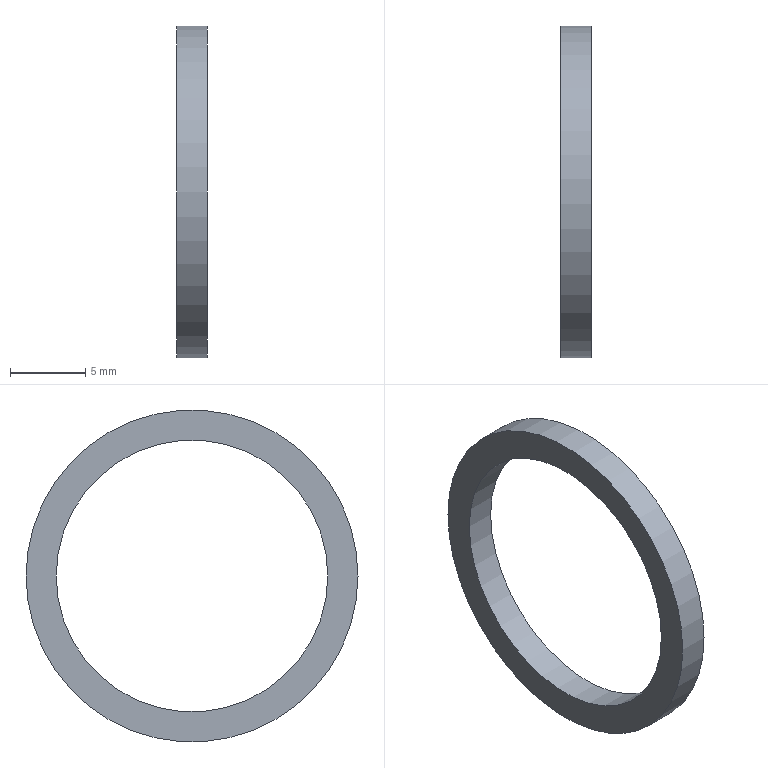Component | NX | PISTON_RING | 1 solid | 4 faces | box 2 x 22 x 22 mm | volume 251 mm3 | cylinder 2 | plane 2 | commonest cylinder face diameters 22 x1 18 x1
STEP:
#1=CARTESIAN_POINT('',(0.,0.,0.));
#2=DIRECTION('',(0.,0.,1.));
#3=DIRECTION('',(1.,0.,0.));
#4=AXIS2_PLACEMENT_3D('',#1,#2,#3);
#5=CARTESIAN_POINT('',(-119.54,-11.,18.5));
#6=VERTEX_POINT('',#5);
#7=CARTESIAN_POINT('',(-119.54,-22.,18.5));
#8=DIRECTION('',(1.,0.,0.));
#9=DIRECTION('',(0.,1.,0.));
#10=AXIS2_PLACEMENT_3D('',#7,#8,#9);
#11=CIRCLE('',#10,11.);
#12=CARTESIAN_POINT('',(-119.54,-22.,18.5));
#13=DIRECTION('',(1.,0.,0.));
#14=DIRECTION('',(0.,-1.,0.));
#15=AXIS2_PLACEMENT_3D('',#12,#13,#14);
#16=CYLINDRICAL_SURFACE('',#15,11.);
#17=CARTESIAN_POINT('',(3.142,0.));
#18=DIRECTION('',(1.,0.));
#19=VECTOR('',#18,1.);
#20=LINE('',#17,#19);
#21=(GEOMETRIC_REPRESENTATION_CONTEXT(2)PARAMETRIC_REPRESENTATION_CONTEXT()REPRESENTATION_CONTEXT('',''));
#22=DEFINITIONAL_REPRESENTATION('',(#20),#21);
#23=PCURVE('',#16,#22);
#24=CARTESIAN_POINT('',(-119.54,-22.,18.5));
#25=DIRECTION('',(1.,0.,0.));
#26=DIRECTION('',(0.,-1.,0.));
#27=AXIS2_PLACEMENT_3D('',#24,#25,#26);
#28=PLANE('',#27);
#29=CARTESIAN_POINT('',(0.,0.));
#30=DIRECTION('',(-1.,0.));
#31=AXIS2_PLACEMENT_2D('',#29,#30);
#32=CIRCLE('',#31,11.);
#33=(GEOMETRIC_REPRESENTATION_CONTEXT(2)PARAMETRIC_REPRESENTATION_CONTEXT()REPRESENTATION_CONTEXT('',''));
#34=DEFINITIONAL_REPRESENTATION('',(#32),#33);
#35=PCURVE('',#28,#34);
#36=SURFACE_CURVE('',#11,(#23,#35),.PCURVE_S1.);
#37=EDGE_CURVE('',#6,#6,#36,.T.);
#38=ORIENTED_EDGE('',*,*,#37,.T.);
#39=CARTESIAN_POINT('',(-117.54,-11.,18.5));
#40=VERTEX_POINT('',#39);
#41=CARTESIAN_POINT('',(-119.54,-11.,18.5));
#42=CARTESIAN_POINT('',(-117.54,-11.,18.5));
#43=B_SPLINE_CURVE_WITH_KNOTS('',1,(#41,#42),.UNSPECIFIED.,.F.,.F.,(2,2),(0.,2.),.PIECEWISE_BEZIER_KNOTS.);
#44=CARTESIAN_POINT('',(9.425,0.));
#45=DIRECTION('',(0.,1.));
#46=VECTOR('',#45,1.);
#47=LINE('',#44,#46);
#48=(GEOMETRIC_REPRESENTATION_CONTEXT(2)PARAMETRIC_REPRESENTATION_CONTEXT()REPRESENTATION_CONTEXT('',''));
#49=DEFINITIONAL_REPRESENTATION('',(#47),#48);
#50=PCURVE('',#16,#49);
#51=CARTESIAN_POINT('',(3.142,0.));
#52=DIRECTION('',(0.,1.));
#53=VECTOR('',#52,1.);
#54=LINE('',#51,#53);
#55=(GEOMETRIC_REPRESENTATION_CONTEXT(2)PARAMETRIC_REPRESENTATION_CONTEXT()REPRESENTATION_CONTEXT('',''));
#56=DEFINITIONAL_REPRESENTATION('',(#54),#55);
#57=PCURVE('',#16,#56);
#58=SEAM_CURVE('',#43,(#50,#57),.PCURVE_S1.);
#59=EDGE_CURVE('',#6,#40,#58,.T.);
#60=ORIENTED_EDGE('',*,*,#59,.T.);
#61=CARTESIAN_POINT('',(-117.54,-22.,18.5));
#62=DIRECTION('',(1.,0.,0.));
#63=DIRECTION('',(0.,1.,0.));
#64=AXIS2_PLACEMENT_3D('',#61,#62,#63);
#65=CIRCLE('',#64,11.);
#66=CARTESIAN_POINT('',(3.142,2.));
#67=DIRECTION('',(1.,0.));
#68=VECTOR('',#67,1.);
#69=LINE('',#66,#68);
#70=(GEOMETRIC_REPRESENTATION_CONTEXT(2)PARAMETRIC_REPRESENTATION_CONTEXT()REPRESENTATION_CONTEXT('',''));
#71=DEFINITIONAL_REPRESENTATION('',(#69),#70);
#72=PCURVE('',#16,#71);
#73=CARTESIAN_POINT('',(-117.54,-22.,18.5));
#74=DIRECTION('',(1.,0.,0.));
#75=DIRECTION('',(0.,-1.,0.));
#76=AXIS2_PLACEMENT_3D('',#73,#74,#75);
#77=PLANE('',#76);
#78=CARTESIAN_POINT('',(0.,0.));
#79=DIRECTION('',(-1.,0.));
#80=AXIS2_PLACEMENT_2D('',#78,#79);
#81=CIRCLE('',#80,11.);
#82=(GEOMETRIC_REPRESENTATION_CONTEXT(2)PARAMETRIC_REPRESENTATION_CONTEXT()REPRESENTATION_CONTEXT('',''));
#83=DEFINITIONAL_REPRESENTATION('',(#81),#82);
#84=PCURVE('',#77,#83);
#85=SURFACE_CURVE('',#65,(#72,#84),.PCURVE_S1.);
#86=EDGE_CURVE('',#40,#40,#85,.T.);
#87=ORIENTED_EDGE('',*,*,#86,.F.);
#88=ORIENTED_EDGE('',*,*,#59,.F.);
#89=EDGE_LOOP('',(#38,#60,#87,#88));
#90=FACE_BOUND('',#89,.T.);
#91=ADVANCED_FACE('',(#90),#16,.T.);
#92=CARTESIAN_POINT('',(-119.54,-13.,18.5));
#93=VERTEX_POINT('',#92);
#94=CARTESIAN_POINT('',(-119.54,-22.,18.5));
#95=DIRECTION('',(1.,0.,0.));
#96=DIRECTION('',(0.,1.,0.));
#97=AXIS2_PLACEMENT_3D('',#94,#95,#96);
#98=CIRCLE('',#97,9.);
#99=CARTESIAN_POINT('',(-119.54,-22.,18.5));
#100=DIRECTION('',(1.,0.,0.));
#101=DIRECTION('',(0.,-1.,0.));
#102=AXIS2_PLACEMENT_3D('',#99,#100,#101);
#103=CYLINDRICAL_SURFACE('',#102,9.);
#104=CARTESIAN_POINT('',(3.142,0.));
#105=DIRECTION('',(1.,0.));
#106=VECTOR('',#105,1.);
#107=LINE('',#104,#106);
#108=(GEOMETRIC_REPRESENTATION_CONTEXT(2)PARAMETRIC_REPRESENTATION_CONTEXT()REPRESENTATION_CONTEXT('',''));
#109=DEFINITIONAL_REPRESENTATION('',(#107),#108);
#110=PCURVE('',#103,#109);
#111=CARTESIAN_POINT('',(0.,0.));
#112=DIRECTION('',(-1.,0.));
#113=AXIS2_PLACEMENT_2D('',#111,#112);
#114=CIRCLE('',#113,9.);
#115=(GEOMETRIC_REPRESENTATION_CONTEXT(2)PARAMETRIC_REPRESENTATION_CONTEXT()REPRESENTATION_CONTEXT('',''));
#116=DEFINITIONAL_REPRESENTATION('',(#114),#115);
#117=PCURVE('',#28,#116);
#118=SURFACE_CURVE('',#98,(#110,#117),.PCURVE_S1.);
#119=EDGE_CURVE('',#93,#93,#118,.T.);
#120=ORIENTED_EDGE('',*,*,#119,.T.);
#121=CARTESIAN_POINT('',(-117.54,-13.,18.5));
#122=VERTEX_POINT('',#121);
#123=CARTESIAN_POINT('',(-119.54,-13.,18.5));
#124=CARTESIAN_POINT('',(-117.54,-13.,18.5));
#125=B_SPLINE_CURVE_WITH_KNOTS('',1,(#123,#124),.UNSPECIFIED.,.F.,.F.,(2,2),(0.,2.),.PIECEWISE_BEZIER_KNOTS.);
#126=CARTESIAN_POINT('',(9.425,0.));
#127=DIRECTION('',(0.,1.));
#128=VECTOR('',#127,1.);
#129=LINE('',#126,#128);
#130=(GEOMETRIC_REPRESENTATION_CONTEXT(2)PARAMETRIC_REPRESENTATION_CONTEXT()REPRESENTATION_CONTEXT('',''));
#131=DEFINITIONAL_REPRESENTATION('',(#129),#130);
#132=PCURVE('',#103,#131);
#133=CARTESIAN_POINT('',(3.142,0.));
#134=DIRECTION('',(0.,1.));
#135=VECTOR('',#134,1.);
#136=LINE('',#133,#135);
#137=(GEOMETRIC_REPRESENTATION_CONTEXT(2)PARAMETRIC_REPRESENTATION_CONTEXT()REPRESENTATION_CONTEXT('',''));
#138=DEFINITIONAL_REPRESENTATION('',(#136),#137);
#139=PCURVE('',#103,#138);
#140=SEAM_CURVE('',#125,(#132,#139),.PCURVE_S1.);
#141=EDGE_CURVE('',#93,#122,#140,.T.);
#142=ORIENTED_EDGE('',*,*,#141,.T.);
#143=CARTESIAN_POINT('',(-117.54,-22.,18.5));
#144=DIRECTION('',(1.,0.,0.));
#145=DIRECTION('',(0.,1.,0.));
#146=AXIS2_PLACEMENT_3D('',#143,#144,#145);
#147=CIRCLE('',#146,9.);
#148=CARTESIAN_POINT('',(3.142,2.));
#149=DIRECTION('',(1.,0.));
#150=VECTOR('',#149,1.);
#151=LINE('',#148,#150);
#152=(GEOMETRIC_REPRESENTATION_CONTEXT(2)PARAMETRIC_REPRESENTATION_CONTEXT()REPRESENTATION_CONTEXT('',''));
#153=DEFINITIONAL_REPRESENTATION('',(#151),#152);
#154=PCURVE('',#103,#153);
#155=CARTESIAN_POINT('',(0.,0.));
#156=DIRECTION('',(-1.,0.));
#157=AXIS2_PLACEMENT_2D('',#155,#156);
#158=CIRCLE('',#157,9.);
#159=(GEOMETRIC_REPRESENTATION_CONTEXT(2)PARAMETRIC_REPRESENTATION_CONTEXT()REPRESENTATION_CONTEXT('',''));
#160=DEFINITIONAL_REPRESENTATION('',(#158),#159);
#161=PCURVE('',#77,#160);
#162=SURFACE_CURVE('',#147,(#154,#161),.PCURVE_S1.);
#163=EDGE_CURVE('',#122,#122,#162,.T.);
#164=ORIENTED_EDGE('',*,*,#163,.F.);
#165=ORIENTED_EDGE('',*,*,#141,.F.);
#166=EDGE_LOOP('',(#120,#142,#164,#165));
#167=FACE_BOUND('',#166,.F.);
#168=ADVANCED_FACE('',(#167),#103,.F.);
#169=ORIENTED_EDGE('',*,*,#37,.F.);
#170=EDGE_LOOP('',(#169));
#171=FACE_BOUND('',#170,.T.);
#172=ORIENTED_EDGE('',*,*,#119,.T.);
#173=EDGE_LOOP('',(#172));
#174=FACE_BOUND('',#173,.T.);
#175=ADVANCED_FACE('',(#171,#174),#28,.F.);
#176=ORIENTED_EDGE('',*,*,#86,.T.);
#177=EDGE_LOOP('',(#176));
#178=FACE_BOUND('',#177,.T.);
#179=ORIENTED_EDGE('',*,*,#163,.F.);
#180=EDGE_LOOP('',(#179));
#181=FACE_BOUND('',#180,.T.);
#182=ADVANCED_FACE('',(#178,#181),#77,.T.);
#183=CLOSED_SHELL('',(#91,#168,#175,#182));
#184=MANIFOLD_SOLID_BREP('',#183);
#185=(LENGTH_UNIT()NAMED_UNIT(*)SI_UNIT(.MILLI.,.METRE.));
#186=UNCERTAINTY_MEASURE_WITH_UNIT(LENGTH_MEASURE(0.00001),#185,'','');
#187=(NAMED_UNIT(*)PLANE_ANGLE_UNIT()SI_UNIT($,.RADIAN.));
#188=(NAMED_UNIT(*)SI_UNIT($,.STERADIAN.)SOLID_ANGLE_UNIT());
#189=(GEOMETRIC_REPRESENTATION_CONTEXT(3)GLOBAL_UNCERTAINTY_ASSIGNED_CONTEXT((#186))GLOBAL_UNIT_ASSIGNED_CONTEXT((#185,#187,#188))REPRESENTATION_CONTEXT('',''));
#190=ADVANCED_BREP_SHAPE_REPRESENTATION('',(#4,#184),#189);